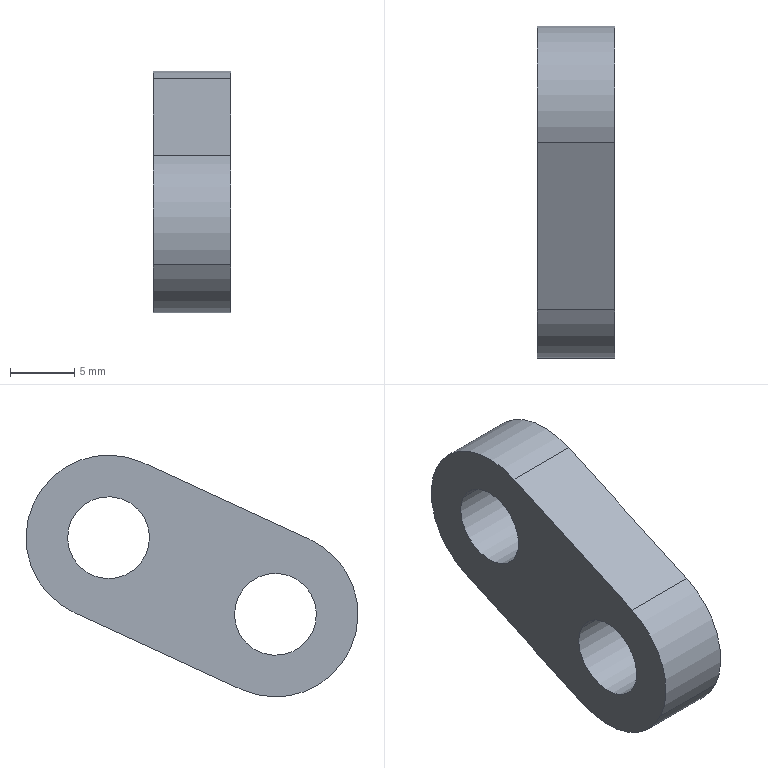Component | SolidWorks | AD12-MC01H-4_2_03.SDASM-1_AD12-_MC01H-4_c.sdprt-1 | 1 solid | 11 faces | box 6 x 25.75 x 18.75 mm | volume 1486 mm3 | cylinder 7 | plane 4 | commonest cylinder face diameters 6.35 x4 12.8 x3
STEP:
#1=COLOUR_RGB('',0.7922,0.8196,0.9333);
#2=FILL_AREA_STYLE_COLOUR('',#1);
#3=FILL_AREA_STYLE('',(#2));
#4=SURFACE_STYLE_FILL_AREA(#3);
#5=SURFACE_SIDE_STYLE('',(#4));
#6=SURFACE_STYLE_USAGE(.BOTH.,#5);
#7=PRESENTATION_STYLE_ASSIGNMENT((#6));
#8=CARTESIAN_POINT('',(-12.398,-10.,13.398));
#9=VERTEX_POINT('',#8);
#10=CARTESIAN_POINT('',(-12.398,-9.773,13.502));
#11=VERTEX_POINT('',#10);
#12=CARTESIAN_POINT('',(-12.398,-9.886,13.45));
#13=DIRECTION('',(1.,0.,0.));
#14=DIRECTION('',(0.,0.9087,0.4176));
#15=AXIS2_PLACEMENT_3D('',#12,#13,#14);
#16=CIRCLE('',#15,0.125);
#17=EDGE_CURVE('',#9,#11,#16,.T.);
#18=ORIENTED_EDGE('',*,*,#17,.F.);
#19=CARTESIAN_POINT('',(-12.162,-10.,13.398));
#20=VERTEX_POINT('',#19);
#21=CARTESIAN_POINT('',(-12.398,-10.,13.398));
#22=DIRECTION('',(1.,0.,0.));
#23=VECTOR('',#22,39.37);
#24=LINE('',#21,#23);
#25=EDGE_CURVE('',#9,#20,#24,.T.);
#26=ORIENTED_EDGE('',*,*,#25,.T.);
#27=CARTESIAN_POINT('',(-12.162,-9.773,13.502));
#28=VERTEX_POINT('',#27);
#29=CARTESIAN_POINT('',(-12.162,-9.886,13.45));
#30=DIRECTION('',(-1.,0.,0.));
#31=DIRECTION('',(0.,0.9087,0.4176));
#32=AXIS2_PLACEMENT_3D('',#29,#30,#31);
#33=CIRCLE('',#32,0.125);
#34=EDGE_CURVE('',#28,#20,#33,.T.);
#35=ORIENTED_EDGE('',*,*,#34,.F.);
#36=CARTESIAN_POINT('',(-12.398,-9.773,13.502));
#37=DIRECTION('',(1.,0.,0.));
#38=VECTOR('',#37,39.37);
#39=LINE('',#36,#38);
#40=EDGE_CURVE('',#11,#28,#39,.T.);
#41=ORIENTED_EDGE('',*,*,#40,.F.);
#42=EDGE_LOOP('',(#18,#26,#35,#41));
#43=FACE_OUTER_BOUND('',#42,.T.);
#44=CARTESIAN_POINT('',(-12.398,-9.886,13.45));
#45=DIRECTION('',(1.,0.,0.));
#46=DIRECTION('',(0.,0.9087,0.4176));
#47=AXIS2_PLACEMENT_3D('',#44,#45,#46);
#48=CYLINDRICAL_SURFACE('',#47,0.125);
#49=ADVANCED_FACE('',(#43),#48,.F.);
#50=CARTESIAN_POINT('',(-12.162,-9.781,13.221));
#51=VERTEX_POINT('',#50);
#52=CARTESIAN_POINT('',(-12.162,-10.115,13.345));
#53=VERTEX_POINT('',#52);
#54=CARTESIAN_POINT('',(-12.162,-9.886,13.45));
#55=DIRECTION('',(-1.,0.,0.));
#56=DIRECTION('',(0.,-0.9087,-0.4176));
#57=AXIS2_PLACEMENT_3D('',#54,#55,#56);
#58=CIRCLE('',#57,0.252);
#59=EDGE_CURVE('',#51,#53,#58,.T.);
#60=ORIENTED_EDGE('',*,*,#59,.T.);
#61=CARTESIAN_POINT('',(-12.398,-10.115,13.345));
#62=VERTEX_POINT('',#61);
#63=CARTESIAN_POINT('',(-12.398,-10.115,13.345));
#64=DIRECTION('',(-1.,0.,0.));
#65=VECTOR('',#64,39.37);
#66=LINE('',#63,#65);
#67=EDGE_CURVE('',#53,#62,#66,.T.);
#68=ORIENTED_EDGE('',*,*,#67,.T.);
#69=CARTESIAN_POINT('',(-12.398,-9.781,13.221));
#70=VERTEX_POINT('',#69);
#71=CARTESIAN_POINT('',(-12.398,-9.886,13.45));
#72=DIRECTION('',(-1.,0.,0.));
#73=DIRECTION('',(0.,-0.9087,-0.4176));
#74=AXIS2_PLACEMENT_3D('',#71,#72,#73);
#75=CIRCLE('',#74,0.252);
#76=EDGE_CURVE('',#70,#62,#75,.T.);
#77=ORIENTED_EDGE('',*,*,#76,.F.);
#78=CARTESIAN_POINT('',(-12.398,-9.781,13.221));
#79=DIRECTION('',(1.,0.,0.));
#80=VECTOR('',#79,39.37);
#81=LINE('',#78,#80);
#82=EDGE_CURVE('',#70,#51,#81,.T.);
#83=ORIENTED_EDGE('',*,*,#82,.T.);
#84=EDGE_LOOP('',(#60,#68,#77,#83));
#85=FACE_OUTER_BOUND('',#84,.T.);
#86=CARTESIAN_POINT('',(-12.398,-9.886,13.45));
#87=DIRECTION('',(-1.,0.,0.));
#88=DIRECTION('',(0.,-0.9087,-0.4176));
#89=AXIS2_PLACEMENT_3D('',#86,#87,#88);
#90=CYLINDRICAL_SURFACE('',#89,0.252);
#91=ADVANCED_FACE('',(#85),#90,.T.);
#92=CARTESIAN_POINT('',(-12.398,-9.49,13.632));
#93=VERTEX_POINT('',#92);
#94=CARTESIAN_POINT('',(-12.398,-9.263,13.737));
#95=VERTEX_POINT('',#94);
#96=CARTESIAN_POINT('',(-12.398,-9.376,13.685));
#97=DIRECTION('',(1.,0.,0.));
#98=DIRECTION('',(0.,0.9087,0.4176));
#99=AXIS2_PLACEMENT_3D('',#96,#97,#98);
#100=CIRCLE('',#99,0.125);
#101=EDGE_CURVE('',#93,#95,#100,.T.);
#102=ORIENTED_EDGE('',*,*,#101,.F.);
#103=CARTESIAN_POINT('',(-12.162,-9.49,13.632));
#104=VERTEX_POINT('',#103);
#105=CARTESIAN_POINT('',(-12.398,-9.49,13.632));
#106=DIRECTION('',(1.,0.,0.));
#107=VECTOR('',#106,39.37);
#108=LINE('',#105,#107);
#109=EDGE_CURVE('',#93,#104,#108,.T.);
#110=ORIENTED_EDGE('',*,*,#109,.T.);
#111=CARTESIAN_POINT('',(-12.162,-9.263,13.737));
#112=VERTEX_POINT('',#111);
#113=CARTESIAN_POINT('',(-12.162,-9.376,13.685));
#114=DIRECTION('',(-1.,0.,0.));
#115=DIRECTION('',(0.,0.9087,0.4176));
#116=AXIS2_PLACEMENT_3D('',#113,#114,#115);
#117=CIRCLE('',#116,0.125);
#118=EDGE_CURVE('',#112,#104,#117,.T.);
#119=ORIENTED_EDGE('',*,*,#118,.F.);
#120=CARTESIAN_POINT('',(-12.398,-9.263,13.737));
#121=DIRECTION('',(1.,0.,0.));
#122=VECTOR('',#121,39.37);
#123=LINE('',#120,#122);
#124=EDGE_CURVE('',#95,#112,#123,.T.);
#125=ORIENTED_EDGE('',*,*,#124,.F.);
#126=EDGE_LOOP('',(#102,#110,#119,#125));
#127=FACE_OUTER_BOUND('',#126,.T.);
#128=CARTESIAN_POINT('',(-12.398,-9.376,13.685));
#129=DIRECTION('',(1.,0.,0.));
#130=DIRECTION('',(0.,0.9087,0.4176));
#131=AXIS2_PLACEMENT_3D('',#128,#129,#130);
#132=CYLINDRICAL_SURFACE('',#131,0.125);
#133=ADVANCED_FACE('',(#127),#132,.F.);
#134=CARTESIAN_POINT('',(-12.398,-9.886,13.45));
#135=DIRECTION('',(1.,0.,0.));
#136=DIRECTION('',(0.,0.9087,0.4176));
#137=AXIS2_PLACEMENT_3D('',#134,#135,#136);
#138=CIRCLE('',#137,0.125);
#139=EDGE_CURVE('',#11,#9,#138,.T.);
#140=ORIENTED_EDGE('',*,*,#139,.T.);
#141=ORIENTED_EDGE('',*,*,#17,.T.);
#142=EDGE_LOOP('',(#140,#141));
#143=FACE_BOUND('',#142,.T.);
#144=CARTESIAN_POINT('',(-12.398,-9.271,13.456));
#145=VERTEX_POINT('',#144);
#146=CARTESIAN_POINT('',(-12.398,-9.271,13.456));
#147=DIRECTION('',(0.,-0.9087,-0.4176));
#148=VECTOR('',#147,39.37);
#149=LINE('',#146,#148);
#150=EDGE_CURVE('',#145,#70,#149,.T.);
#151=ORIENTED_EDGE('',*,*,#150,.T.);
#152=ORIENTED_EDGE('',*,*,#76,.T.);
#153=CARTESIAN_POINT('',(-12.398,-9.991,13.679));
#154=VERTEX_POINT('',#153);
#155=CARTESIAN_POINT('',(-12.398,-9.886,13.45));
#156=DIRECTION('',(-1.,0.,0.));
#157=DIRECTION('',(0.,-0.9087,-0.4176));
#158=AXIS2_PLACEMENT_3D('',#155,#156,#157);
#159=CIRCLE('',#158,0.252);
#160=EDGE_CURVE('',#62,#154,#159,.T.);
#161=ORIENTED_EDGE('',*,*,#160,.T.);
#162=CARTESIAN_POINT('',(-12.398,-9.482,13.913));
#163=VERTEX_POINT('',#162);
#164=CARTESIAN_POINT('',(-12.398,-9.482,13.913));
#165=DIRECTION('',(0.,0.9087,0.4176));
#166=VECTOR('',#165,39.37);
#167=LINE('',#164,#166);
#168=EDGE_CURVE('',#154,#163,#167,.T.);
#169=ORIENTED_EDGE('',*,*,#168,.T.);
#170=CARTESIAN_POINT('',(-12.398,-9.376,13.685));
#171=DIRECTION('',(-1.,0.,0.));
#172=DIRECTION('',(0.,-0.9087,-0.4176));
#173=AXIS2_PLACEMENT_3D('',#170,#171,#172);
#174=CIRCLE('',#173,0.252);
#175=EDGE_CURVE('',#163,#145,#174,.T.);
#176=ORIENTED_EDGE('',*,*,#175,.T.);
#177=EDGE_LOOP('',(#151,#152,#161,#169,#176));
#178=FACE_OUTER_BOUND('',#177,.T.);
#179=CARTESIAN_POINT('',(-12.398,-9.376,13.685));
#180=DIRECTION('',(1.,0.,0.));
#181=DIRECTION('',(0.,0.9087,0.4176));
#182=AXIS2_PLACEMENT_3D('',#179,#180,#181);
#183=CIRCLE('',#182,0.125);
#184=EDGE_CURVE('',#95,#93,#183,.T.);
#185=ORIENTED_EDGE('',*,*,#184,.T.);
#186=ORIENTED_EDGE('',*,*,#101,.T.);
#187=EDGE_LOOP('',(#185,#186));
#188=FACE_BOUND('',#187,.T.);
#189=CARTESIAN_POINT('',(-12.398,-9.376,13.685));
#190=DIRECTION('',(-1.,0.,0.));
#191=DIRECTION('',(0.,-0.9087,-0.4176));
#192=AXIS2_PLACEMENT_3D('',#189,#190,#191);
#193=PLANE('',#192);
#194=ADVANCED_FACE('',(#143,#178,#188),#193,.T.);
#195=ORIENTED_EDGE('',*,*,#25,.F.);
#196=ORIENTED_EDGE('',*,*,#139,.F.);
#197=ORIENTED_EDGE('',*,*,#40,.T.);
#198=CARTESIAN_POINT('',(-12.162,-9.886,13.45));
#199=DIRECTION('',(-1.,0.,0.));
#200=DIRECTION('',(0.,0.9087,0.4176));
#201=AXIS2_PLACEMENT_3D('',#198,#199,#200);
#202=CIRCLE('',#201,0.125);
#203=EDGE_CURVE('',#20,#28,#202,.T.);
#204=ORIENTED_EDGE('',*,*,#203,.F.);
#205=EDGE_LOOP('',(#195,#196,#197,#204));
#206=FACE_OUTER_BOUND('',#205,.T.);
#207=CARTESIAN_POINT('',(-12.398,-9.886,13.45));
#208=DIRECTION('',(1.,0.,0.));
#209=DIRECTION('',(0.,0.9087,0.4176));
#210=AXIS2_PLACEMENT_3D('',#207,#208,#209);
#211=CYLINDRICAL_SURFACE('',#210,0.125);
#212=ADVANCED_FACE('',(#206),#211,.F.);
#213=ORIENTED_EDGE('',*,*,#67,.F.);
#214=CARTESIAN_POINT('',(-12.162,-9.991,13.679));
#215=VERTEX_POINT('',#214);
#216=CARTESIAN_POINT('',(-12.162,-9.886,13.45));
#217=DIRECTION('',(-1.,0.,0.));
#218=DIRECTION('',(0.,-0.9087,-0.4176));
#219=AXIS2_PLACEMENT_3D('',#216,#217,#218);
#220=CIRCLE('',#219,0.252);
#221=EDGE_CURVE('',#53,#215,#220,.T.);
#222=ORIENTED_EDGE('',*,*,#221,.T.);
#223=CARTESIAN_POINT('',(-12.398,-9.991,13.679));
#224=DIRECTION('',(-1.,0.,0.));
#225=VECTOR('',#224,39.37);
#226=LINE('',#223,#225);
#227=EDGE_CURVE('',#215,#154,#226,.T.);
#228=ORIENTED_EDGE('',*,*,#227,.T.);
#229=ORIENTED_EDGE('',*,*,#160,.F.);
#230=EDGE_LOOP('',(#213,#222,#228,#229));
#231=FACE_OUTER_BOUND('',#230,.T.);
#232=CARTESIAN_POINT('',(-12.398,-9.886,13.45));
#233=DIRECTION('',(-1.,0.,0.));
#234=DIRECTION('',(0.,-0.9087,-0.4176));
#235=AXIS2_PLACEMENT_3D('',#232,#233,#234);
#236=CYLINDRICAL_SURFACE('',#235,0.252);
#237=ADVANCED_FACE('',(#231),#236,.T.);
#238=ORIENTED_EDGE('',*,*,#82,.F.);
#239=ORIENTED_EDGE('',*,*,#150,.F.);
#240=CARTESIAN_POINT('',(-12.162,-9.271,13.456));
#241=VERTEX_POINT('',#240);
#242=CARTESIAN_POINT('',(-12.398,-9.271,13.456));
#243=DIRECTION('',(-1.,0.,0.));
#244=VECTOR('',#243,39.37);
#245=LINE('',#242,#244);
#246=EDGE_CURVE('',#241,#145,#245,.T.);
#247=ORIENTED_EDGE('',*,*,#246,.F.);
#248=CARTESIAN_POINT('',(-12.162,-9.271,13.456));
#249=DIRECTION('',(0.,0.9087,0.4176));
#250=VECTOR('',#249,39.37);
#251=LINE('',#248,#250);
#252=EDGE_CURVE('',#51,#241,#251,.T.);
#253=ORIENTED_EDGE('',*,*,#252,.F.);
#254=EDGE_LOOP('',(#238,#239,#247,#253));
#255=FACE_OUTER_BOUND('',#254,.T.);
#256=CARTESIAN_POINT('',(-12.398,-9.271,13.456));
#257=DIRECTION('',(0.,-0.4176,0.9087));
#258=DIRECTION('',(0.,0.9087,0.4176));
#259=AXIS2_PLACEMENT_3D('',#256,#257,#258);
#260=PLANE('',#259);
#261=ADVANCED_FACE('',(#255),#260,.F.);
#262=ORIENTED_EDGE('',*,*,#175,.F.);
#263=CARTESIAN_POINT('',(-12.162,-9.482,13.913));
#264=VERTEX_POINT('',#263);
#265=CARTESIAN_POINT('',(-12.398,-9.482,13.913));
#266=DIRECTION('',(1.,0.,0.));
#267=VECTOR('',#266,39.37);
#268=LINE('',#265,#267);
#269=EDGE_CURVE('',#163,#264,#268,.T.);
#270=ORIENTED_EDGE('',*,*,#269,.T.);
#271=CARTESIAN_POINT('',(-12.162,-9.376,13.685));
#272=DIRECTION('',(-1.,0.,0.));
#273=DIRECTION('',(0.,-0.9087,-0.4176));
#274=AXIS2_PLACEMENT_3D('',#271,#272,#273);
#275=CIRCLE('',#274,0.252);
#276=EDGE_CURVE('',#264,#241,#275,.T.);
#277=ORIENTED_EDGE('',*,*,#276,.T.);
#278=ORIENTED_EDGE('',*,*,#246,.T.);
#279=EDGE_LOOP('',(#262,#270,#277,#278));
#280=FACE_OUTER_BOUND('',#279,.T.);
#281=CARTESIAN_POINT('',(-12.398,-9.376,13.685));
#282=DIRECTION('',(-1.,0.,0.));
#283=DIRECTION('',(0.,-0.9087,-0.4176));
#284=AXIS2_PLACEMENT_3D('',#281,#282,#283);
#285=CYLINDRICAL_SURFACE('',#284,0.252);
#286=ADVANCED_FACE('',(#280),#285,.T.);
#287=ORIENTED_EDGE('',*,*,#269,.F.);
#288=ORIENTED_EDGE('',*,*,#168,.F.);
#289=ORIENTED_EDGE('',*,*,#227,.F.);
#290=CARTESIAN_POINT('',(-12.162,-9.991,13.679));
#291=DIRECTION('',(0.,-0.9087,-0.4176));
#292=VECTOR('',#291,39.37);
#293=LINE('',#290,#292);
#294=EDGE_CURVE('',#264,#215,#293,.T.);
#295=ORIENTED_EDGE('',*,*,#294,.F.);
#296=EDGE_LOOP('',(#287,#288,#289,#295));
#297=FACE_OUTER_BOUND('',#296,.T.);
#298=CARTESIAN_POINT('',(-12.398,-9.991,13.679));
#299=DIRECTION('',(0.,0.4176,-0.9087));
#300=DIRECTION('',(0.,-0.9087,-0.4176));
#301=AXIS2_PLACEMENT_3D('',#298,#299,#300);
#302=PLANE('',#301);
#303=ADVANCED_FACE('',(#297),#302,.F.);
#304=ORIENTED_EDGE('',*,*,#109,.F.);
#305=ORIENTED_EDGE('',*,*,#184,.F.);
#306=ORIENTED_EDGE('',*,*,#124,.T.);
#307=CARTESIAN_POINT('',(-12.162,-9.376,13.685));
#308=DIRECTION('',(-1.,0.,0.));
#309=DIRECTION('',(0.,0.9087,0.4176));
#310=AXIS2_PLACEMENT_3D('',#307,#308,#309);
#311=CIRCLE('',#310,0.125);
#312=EDGE_CURVE('',#104,#112,#311,.T.);
#313=ORIENTED_EDGE('',*,*,#312,.F.);
#314=EDGE_LOOP('',(#304,#305,#306,#313));
#315=FACE_OUTER_BOUND('',#314,.T.);
#316=CARTESIAN_POINT('',(-12.398,-9.376,13.685));
#317=DIRECTION('',(1.,0.,0.));
#318=DIRECTION('',(0.,0.9087,0.4176));
#319=AXIS2_PLACEMENT_3D('',#316,#317,#318);
#320=CYLINDRICAL_SURFACE('',#319,0.125);
#321=ADVANCED_FACE('',(#315),#320,.F.);
#322=ORIENTED_EDGE('',*,*,#34,.T.);
#323=ORIENTED_EDGE('',*,*,#203,.T.);
#324=EDGE_LOOP('',(#322,#323));
#325=FACE_BOUND('',#324,.T.);
#326=ORIENTED_EDGE('',*,*,#59,.F.);
#327=ORIENTED_EDGE('',*,*,#252,.T.);
#328=ORIENTED_EDGE('',*,*,#276,.F.);
#329=ORIENTED_EDGE('',*,*,#294,.T.);
#330=ORIENTED_EDGE('',*,*,#221,.F.);
#331=EDGE_LOOP('',(#326,#327,#328,#329,#330));
#332=FACE_OUTER_BOUND('',#331,.T.);
#333=ORIENTED_EDGE('',*,*,#118,.T.);
#334=ORIENTED_EDGE('',*,*,#312,.T.);
#335=EDGE_LOOP('',(#333,#334));
#336=FACE_BOUND('',#335,.T.);
#337=CARTESIAN_POINT('',(-12.162,-9.376,13.685));
#338=DIRECTION('',(-1.,0.,0.));
#339=DIRECTION('',(0.,-0.9087,-0.4176));
#340=AXIS2_PLACEMENT_3D('',#337,#338,#339);
#341=PLANE('',#340);
#342=ADVANCED_FACE('',(#325,#332,#336),#341,.F.);
#343=CLOSED_SHELL('',(#49,#91,#133,#194,#212,#237,#261,#286,#303,#321,#342));
#344=MANIFOLD_SOLID_BREP('',#343);
#345=STYLED_ITEM('',(#7),#344);
#346=(LENGTH_UNIT()NAMED_UNIT(*)SI_UNIT($,.METRE.));
#347=LENGTH_MEASURE_WITH_UNIT(LENGTH_MEASURE(0.0254),#346);
#348=DIMENSIONAL_EXPONENTS(1.,0.,0.,0.,0.,0.,0.);
#349=(CONVERSION_BASED_UNIT('',#347)LENGTH_UNIT()NAMED_UNIT(#348));
#350=UNCERTAINTY_MEASURE_WITH_UNIT(LENGTH_MEASURE(0.00001),#349,'','');
#351=(NAMED_UNIT(*)PLANE_ANGLE_UNIT()SI_UNIT($,.RADIAN.));
#352=(NAMED_UNIT(*)SI_UNIT($,.STERADIAN.)SOLID_ANGLE_UNIT());
#353=(GEOMETRIC_REPRESENTATION_CONTEXT(3)GLOBAL_UNCERTAINTY_ASSIGNED_CONTEXT((#350))GLOBAL_UNIT_ASSIGNED_CONTEXT((#349,#351,#352))REPRESENTATION_CONTEXT('',''));
#354=MECHANICAL_DESIGN_GEOMETRIC_PRESENTATION_REPRESENTATION('',(#345),#353);
#355=CARTESIAN_POINT('',(0.,0.,0.));
#356=DIRECTION('',(0.,0.,1.));
#357=DIRECTION('',(1.,0.,0.));
#358=AXIS2_PLACEMENT_3D('',#355,#356,#357);
#359=(LENGTH_UNIT()NAMED_UNIT(*)SI_UNIT($,.METRE.));
#360=LENGTH_MEASURE_WITH_UNIT(LENGTH_MEASURE(0.0254),#359);
#361=DIMENSIONAL_EXPONENTS(1.,0.,0.,0.,0.,0.,0.);
#362=(CONVERSION_BASED_UNIT('',#360)LENGTH_UNIT()NAMED_UNIT(#361));
#363=UNCERTAINTY_MEASURE_WITH_UNIT(LENGTH_MEASURE(0.00001),#362,'','');
#364=(NAMED_UNIT(*)PLANE_ANGLE_UNIT()SI_UNIT($,.RADIAN.));
#365=(NAMED_UNIT(*)SI_UNIT($,.STERADIAN.)SOLID_ANGLE_UNIT());
#366=(GEOMETRIC_REPRESENTATION_CONTEXT(3)GLOBAL_UNCERTAINTY_ASSIGNED_CONTEXT((#363))GLOBAL_UNIT_ASSIGNED_CONTEXT((#362,#364,#365))REPRESENTATION_CONTEXT('',''));
#367=ADVANCED_BREP_SHAPE_REPRESENTATION('',(#344,#358),#366);
#368=PRESENTATION_LAYER_ASSIGNMENT('','',(#345));